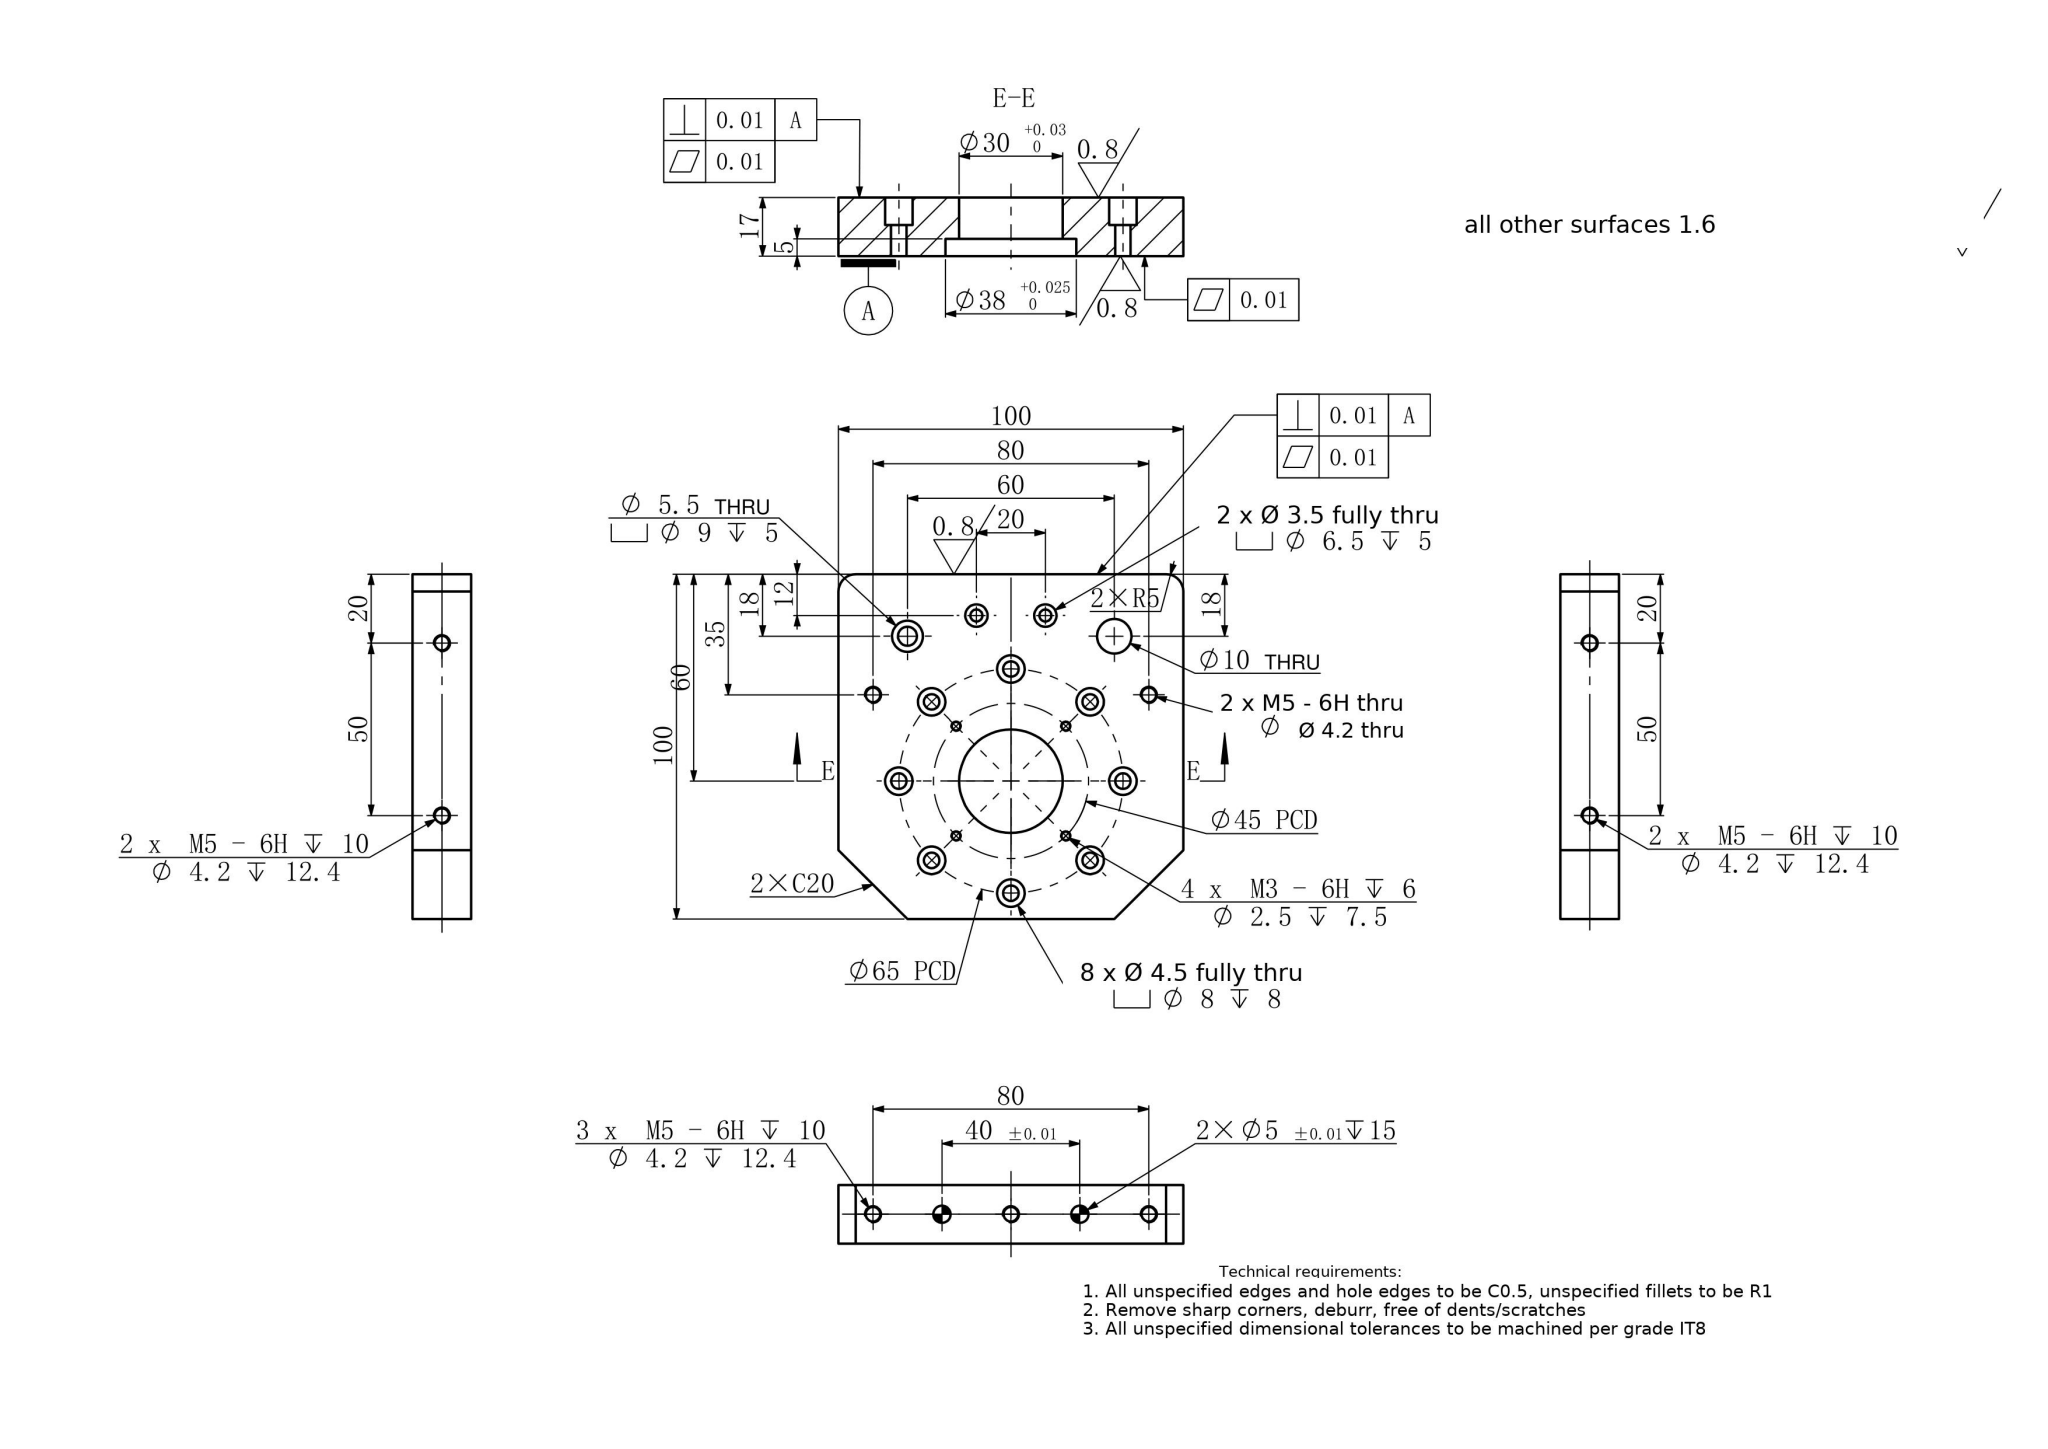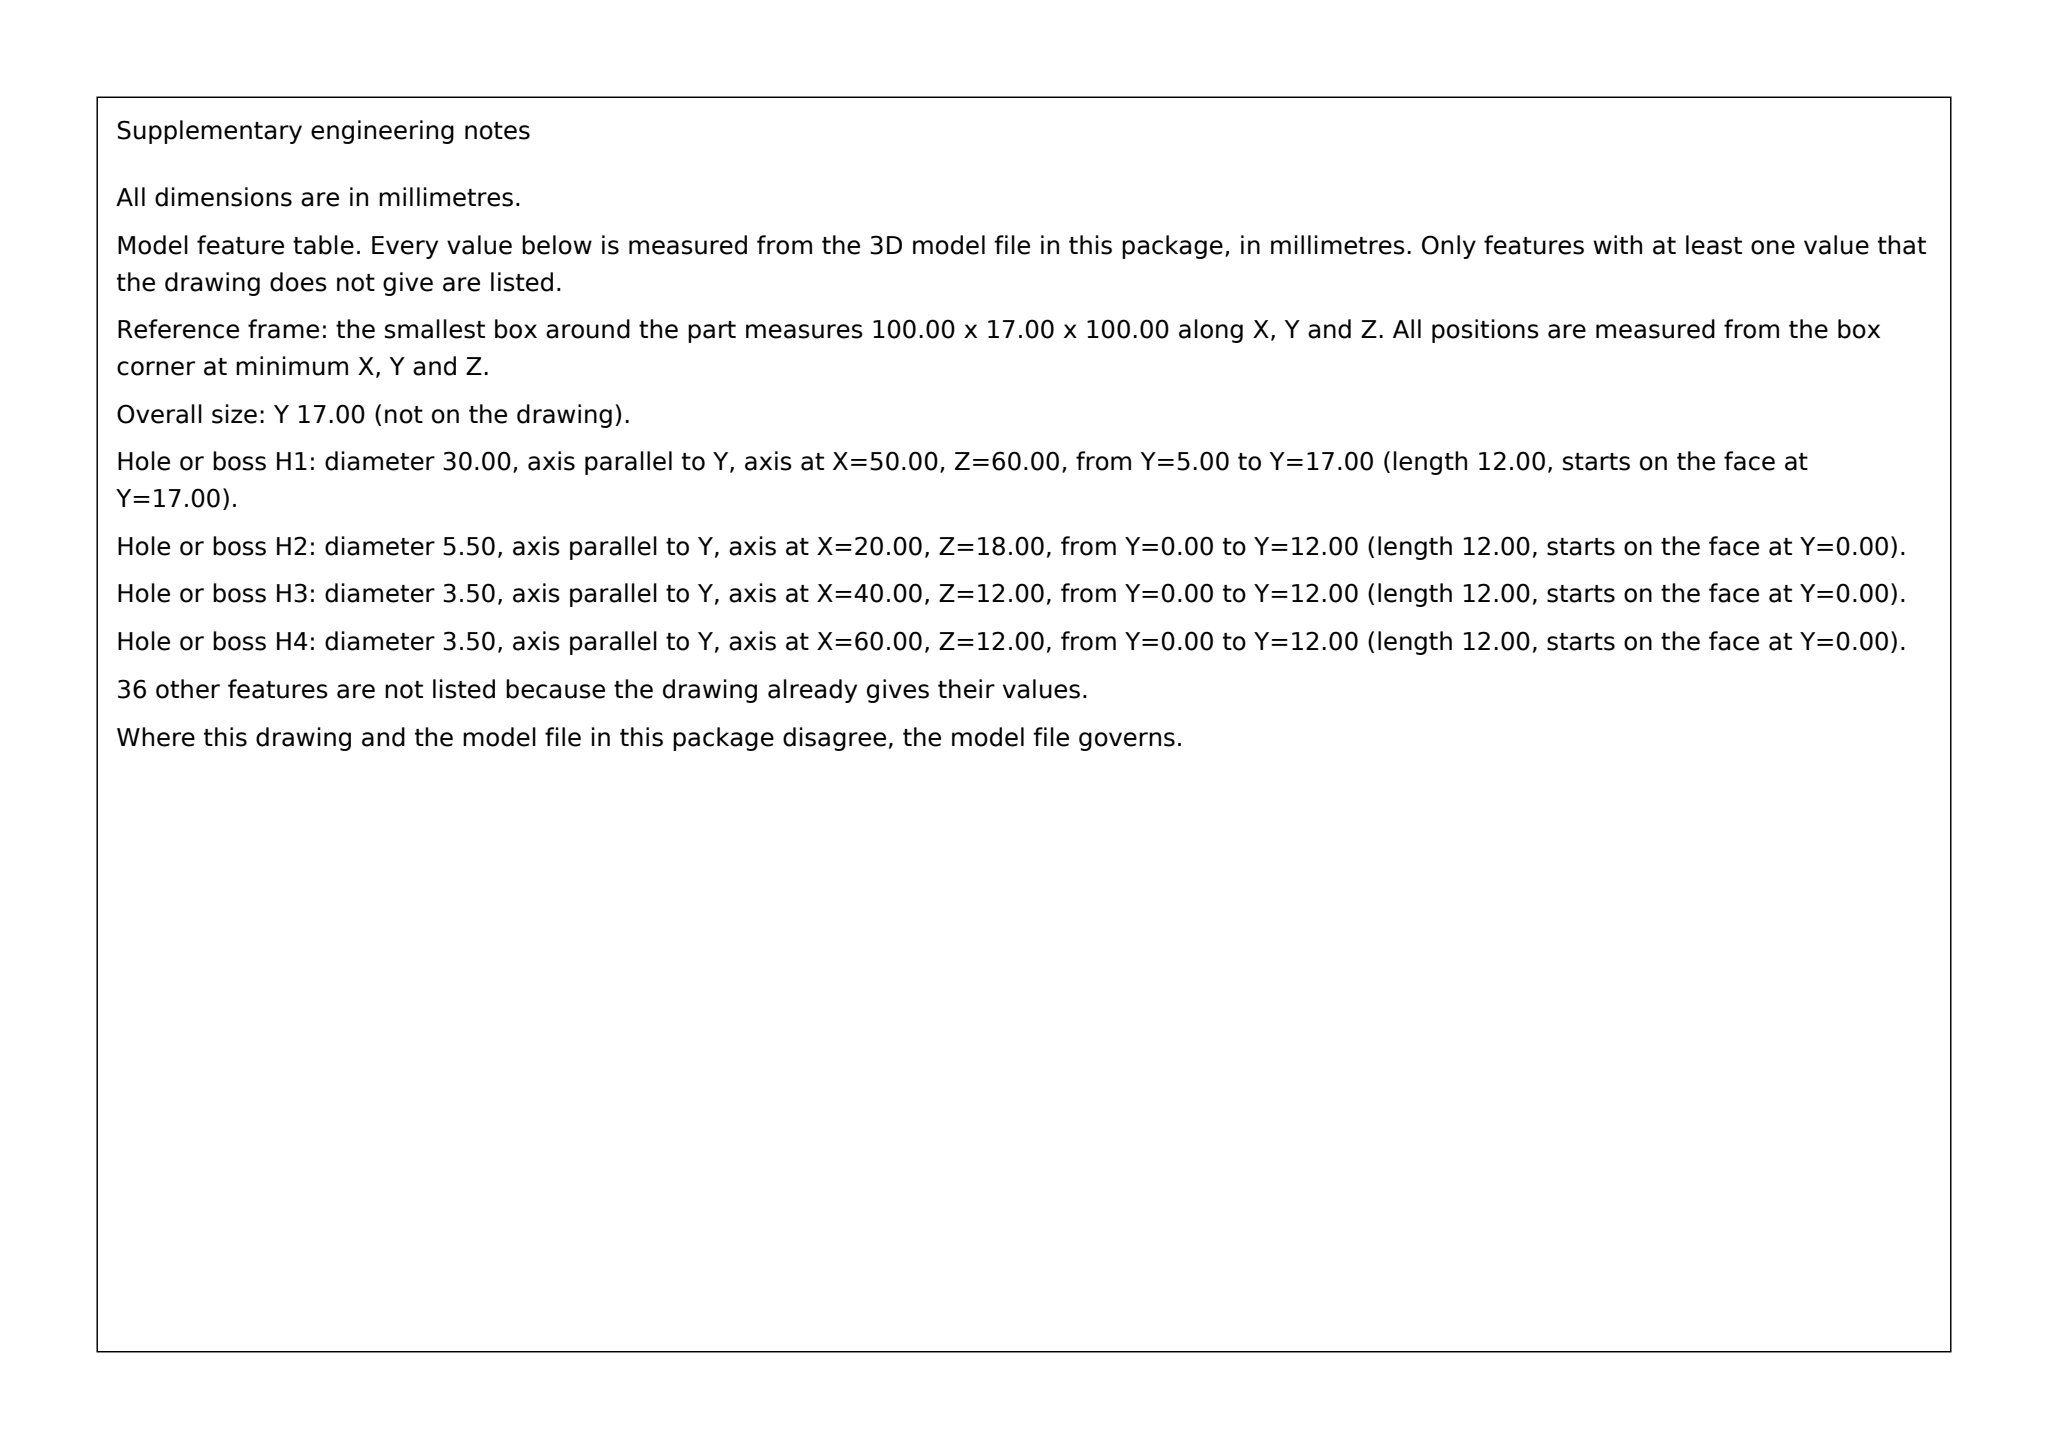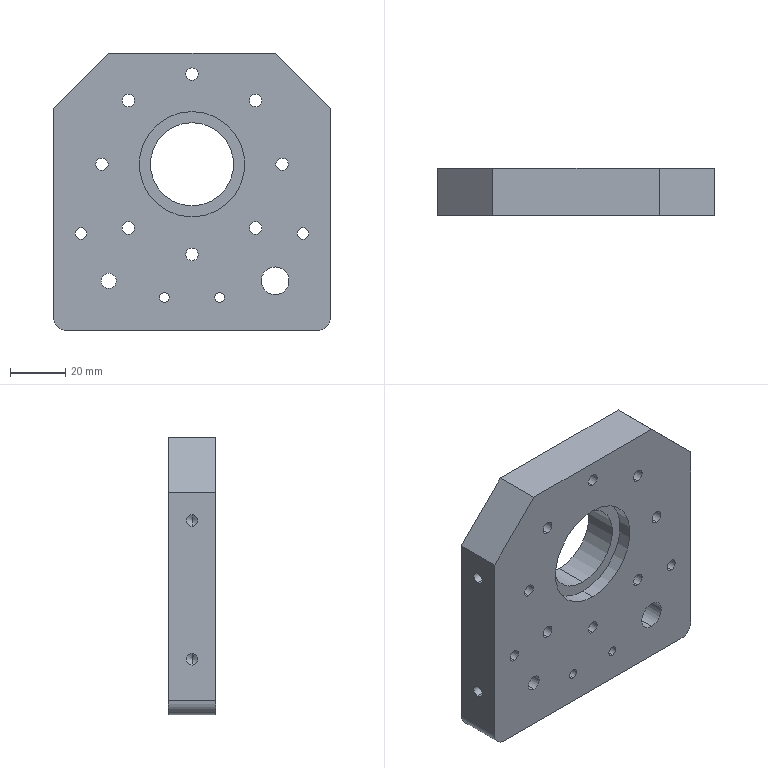Part | SolidWorks | mm | 1 solid | 128 faces | box 100 x 17 x 100 mm | volume 139526 mm3 | cylinder 82 | cone 26 | plane 20 | commonest cylinder face diameters 4.2 x18 8 x16 4.5 x16 2.5 x8 6.5 x4 3.5 x4 5 x4 10 x4
build123d program:
from build123d import *

# Parameters (mm, degrees)
SKETCH1_W                                            = 100
SKETCH1_H                                            = 100
SKETCH1_R                                            = 15
SKETCH1_R_2                                          = 5
BOSS_EXTRUDE1_DEPTH                                  = 8.5
M3_TAPPED_HOLE1_D                                    = 2.5
M3_TAPPED_HOLE1_DEPTH                                = 7.5
M3_TAPPED_HOLE1_TIP                                  = 0.7511
SKETCH4_R                                            = 19
CUT_EXTRUDE1_DEPTH                                   = 5
CYLINDRICAL_COUNTERSUNK_HOLE_1_FOR_M4_HE_D           = 4.5
CYLINDRICAL_COUNTERSUNK_HOLE_1_FOR_M4_HE_CBORE_D     = 8
CYLINDRICAL_COUNTERSUNK_HOLE_1_FOR_M4_HE_CBORE_DEPTH = 8
CIRPATTERN1_COUNT                                    = 8
F_5_0_5_DIAMETER_HOLE1_D                             = 5
F_5_0_5_DIAMETER_HOLE1_DEPTH                         = 15
F_5_0_5_DIAMETER_HOLE1_TIP                           = 1.502
M5_TAPPED_HOLE1_D                                    = 4.2
M5_TAPPED_HOLE1_DEPTH                                = 12.4
M5_TAPPED_HOLE1_TIP                                  = 1.262
M5_TAPPED_HOLE2_D                                    = 4.2
M5_TAPPED_HOLE2_DEPTH                                = 12.4
M5_TAPPED_HOLE2_TIP                                  = 1.262
M5_TAPPED_HOLE3_D                                    = 4.2
M5_TAPPED_HOLE3_DEPTH                                = 12.4
M5_TAPPED_HOLE3_TIP                                  = 1.262
M3_HEX_SOCKET_HEAD_CAP_SCREW_CBORE1_D                = 3.5
M3_HEX_SOCKET_HEAD_CAP_SCREW_CBORE1_CBORE_D          = 6.5
M3_HEX_SOCKET_HEAD_CAP_SCREW_CBORE1_CBORE_DEPTH      = 5
CHAMFER1_SIZE                                        = 20
M5_TAPPED_HOLE4_D                                    = 4.2
CYLINDRICAL_COUNTERSUNK_HOLE_1_FOR_M5_HE_D           = 5.5
CYLINDRICAL_COUNTERSUNK_HOLE_1_FOR_M5_HE_CBORE_D     = 9
CYLINDRICAL_COUNTERSUNK_HOLE_1_FOR_M5_HE_CBORE_DEPTH = 5
FILLET1_R                                            = 5


with BuildPart() as part:
    # Sketch1 → Boss-Extrude1 (new, symmetric)
    with BuildSketch(Plane(origin=(0, 0, 0), x_dir=(1, 0, 0), z_dir=(0, 1, 0))):
        with Locations((0, -50)):
            Rectangle(SKETCH1_W, SKETCH1_H)
        with Locations(Location((0, -60, 0), (0, 0, 270))):
            Circle(SKETCH1_R, mode=Mode.SUBTRACT)
        with Locations(Location((30, -18, 0), (0, 0, 270))):
            Circle(SKETCH1_R_2, mode=Mode.SUBTRACT)
    extrude(amount=BOSS_EXTRUDE1_DEPTH, both=True)

    # M3 Tapped Hole1
    with Locations(Plane(origin=(0, 8.5, 0), x_dir=(1, 0, 0), z_dir=(0, 1, 0))):
        with Locations((-15.91, -44.09), (15.91, -44.09), (15.91, -75.91), (-15.91, -75.91)):
            Hole(M3_TAPPED_HOLE1_D / 2, depth=M3_TAPPED_HOLE1_DEPTH)
            with Locations((0, 0, -(M3_TAPPED_HOLE1_DEPTH + M3_TAPPED_HOLE1_TIP / 2))):  # 118° drill point
                Cone(0, M3_TAPPED_HOLE1_D / 2, M3_TAPPED_HOLE1_TIP, mode=Mode.SUBTRACT)

    # Sketch4 → Cut-Extrude1 (cut)
    with BuildSketch(Plane.XZ.offset(8.5)):
        with Locations(Location((0, 60, 0), (0, 0, 270))):
            Circle(SKETCH4_R)
    extrude(amount=-CUT_EXTRUDE1_DEPTH, mode=Mode.SUBTRACT)

    # Cylindrical Countersunk Hole 1 for M4 He (through all)
    with Locations(Plane(origin=(0, 8.5, 0), x_dir=(1, 0, 0), z_dir=(0, 1, 0))):
        with Locations((-32.5, -60)):
            cylindrical_countersunk_hole_1_for_m4_he = CounterBoreHole(CYLINDRICAL_COUNTERSUNK_HOLE_1_FOR_M4_HE_D / 2, CYLINDRICAL_COUNTERSUNK_HOLE_1_FOR_M4_HE_CBORE_D / 2, CYLINDRICAL_COUNTERSUNK_HOLE_1_FOR_M4_HE_CBORE_DEPTH)

    # CirPattern1: Cylindrical Countersunk Hole 1 for M4 He ×8 about axis
    cirpattern1_axis = Axis((0, 0, 60), (0, 1, 0))
    for i in range(1, CIRPATTERN1_COUNT):
        add(cylindrical_countersunk_hole_1_for_m4_he.rotate(cirpattern1_axis, i * 360 / CIRPATTERN1_COUNT), mode=Mode.SUBTRACT)

    # 5.0 _5_ Diameter Hole1
    with Locations(Plane(origin=(0, 0, 0), x_dir=(-1, 0, 0), z_dir=(0, 0, -1))):
        with Locations((20, 0), (-20, 0)):
            Hole(F_5_0_5_DIAMETER_HOLE1_D / 2, depth=F_5_0_5_DIAMETER_HOLE1_DEPTH)
            with Locations((0, 0, -(F_5_0_5_DIAMETER_HOLE1_DEPTH + F_5_0_5_DIAMETER_HOLE1_TIP / 2))):  # 118° drill point
                Cone(0, F_5_0_5_DIAMETER_HOLE1_D / 2, F_5_0_5_DIAMETER_HOLE1_TIP, mode=Mode.SUBTRACT)

    # M5 Tapped Hole1
    with Locations(Plane(origin=(0, 0, 0), x_dir=(-1, 0, 0), z_dir=(0, 0, -1))):
        with Locations((-40, 0), (40, 0), (0, 0)):
            Hole(M5_TAPPED_HOLE1_D / 2, depth=M5_TAPPED_HOLE1_DEPTH)
            with Locations((0, 0, -(M5_TAPPED_HOLE1_DEPTH + M5_TAPPED_HOLE1_TIP / 2))):  # 118° drill point
                Cone(0, M5_TAPPED_HOLE1_D / 2, M5_TAPPED_HOLE1_TIP, mode=Mode.SUBTRACT)

    # M5 Tapped Hole2
    with Locations(Plane(origin=(50, 0, 0), x_dir=(0, 0, -1), z_dir=(1, 0, 0))):
        with Locations((-20, 0), (-70, 0)):
            Hole(M5_TAPPED_HOLE2_D / 2, depth=M5_TAPPED_HOLE2_DEPTH)
            with Locations((0, 0, -(M5_TAPPED_HOLE2_DEPTH + M5_TAPPED_HOLE2_TIP / 2))):  # 118° drill point
                Cone(0, M5_TAPPED_HOLE2_D / 2, M5_TAPPED_HOLE2_TIP, mode=Mode.SUBTRACT)

    # M5 Tapped Hole3
    with Locations(Plane.ZY.offset(50)):
        with Locations((20, 0), (70, 0)):
            Hole(M5_TAPPED_HOLE3_D / 2, depth=M5_TAPPED_HOLE3_DEPTH)
            with Locations((0, 0, -(M5_TAPPED_HOLE3_DEPTH + M5_TAPPED_HOLE3_TIP / 2))):  # 118° drill point
                Cone(0, M5_TAPPED_HOLE3_D / 2, M5_TAPPED_HOLE3_TIP, mode=Mode.SUBTRACT)

    # M3 Hex Socket Head Cap Screw CBORE1 (through all)
    with Locations(Plane(origin=(0, 8.5, 0), x_dir=(1, 0, 0), z_dir=(0, 1, 0))):
        with Locations((-10, -12), (10, -12)):
            CounterBoreHole(M3_HEX_SOCKET_HEAD_CAP_SCREW_CBORE1_D / 2, M3_HEX_SOCKET_HEAD_CAP_SCREW_CBORE1_CBORE_D / 2, M3_HEX_SOCKET_HEAD_CAP_SCREW_CBORE1_CBORE_DEPTH)

    # Chamfer1
    chamfer1_edges = [part.edges().sort_by_distance(p)[0] for p in [
        (50, 0, 100),
        (-50, 0, 100),
    ]]
    chamfer(chamfer1_edges, length=CHAMFER1_SIZE)

    # M5 Tapped Hole4 (through all)
    with Locations(Plane(origin=(0, 8.5, 0), x_dir=(1, 0, 0), z_dir=(0, 1, 0))):
        with Locations((-40, -35), (40, -35)):
            Hole(M5_TAPPED_HOLE4_D / 2)

    # Cylindrical Countersunk Hole 1 for M5 He (through all)
    with Locations(Plane(origin=(0, 8.5, 0), x_dir=(1, 0, 0), z_dir=(0, 1, 0))):
        with Locations((-30, -18)):
            CounterBoreHole(CYLINDRICAL_COUNTERSUNK_HOLE_1_FOR_M5_HE_D / 2, CYLINDRICAL_COUNTERSUNK_HOLE_1_FOR_M5_HE_CBORE_D / 2, CYLINDRICAL_COUNTERSUNK_HOLE_1_FOR_M5_HE_CBORE_DEPTH)

    # Fillet1
    fillet1_edges = [part.edges().sort_by_distance(p)[0] for p in [
        (-50, 0, 0),
        (50, 0, 0),
    ]]
    fillet(fillet1_edges, radius=FILLET1_R)


solid = part.part